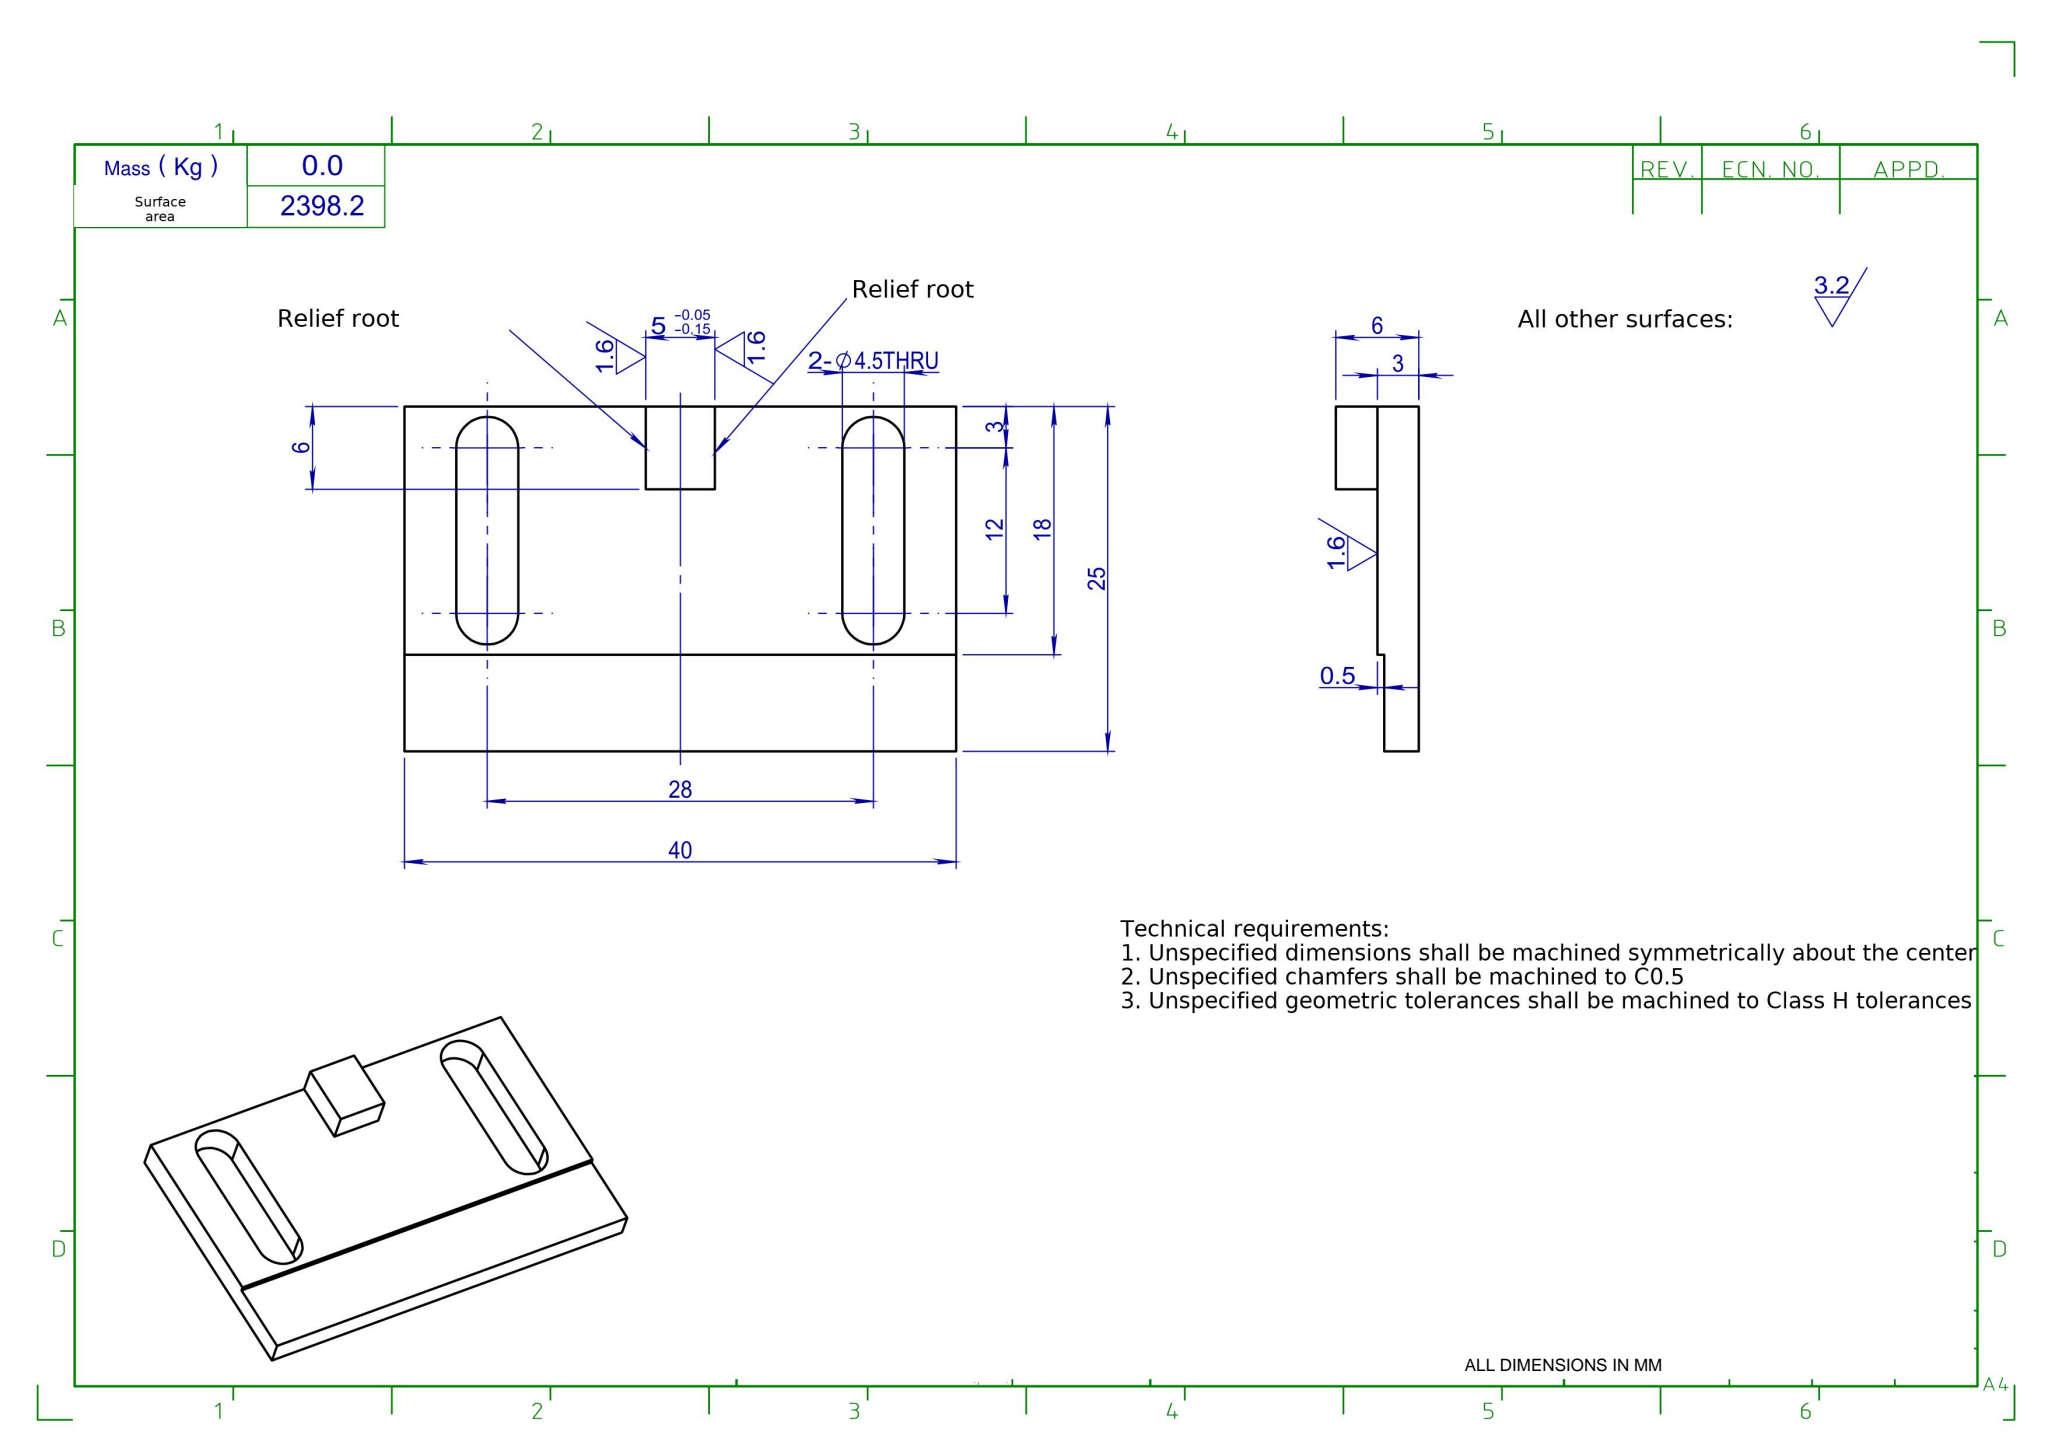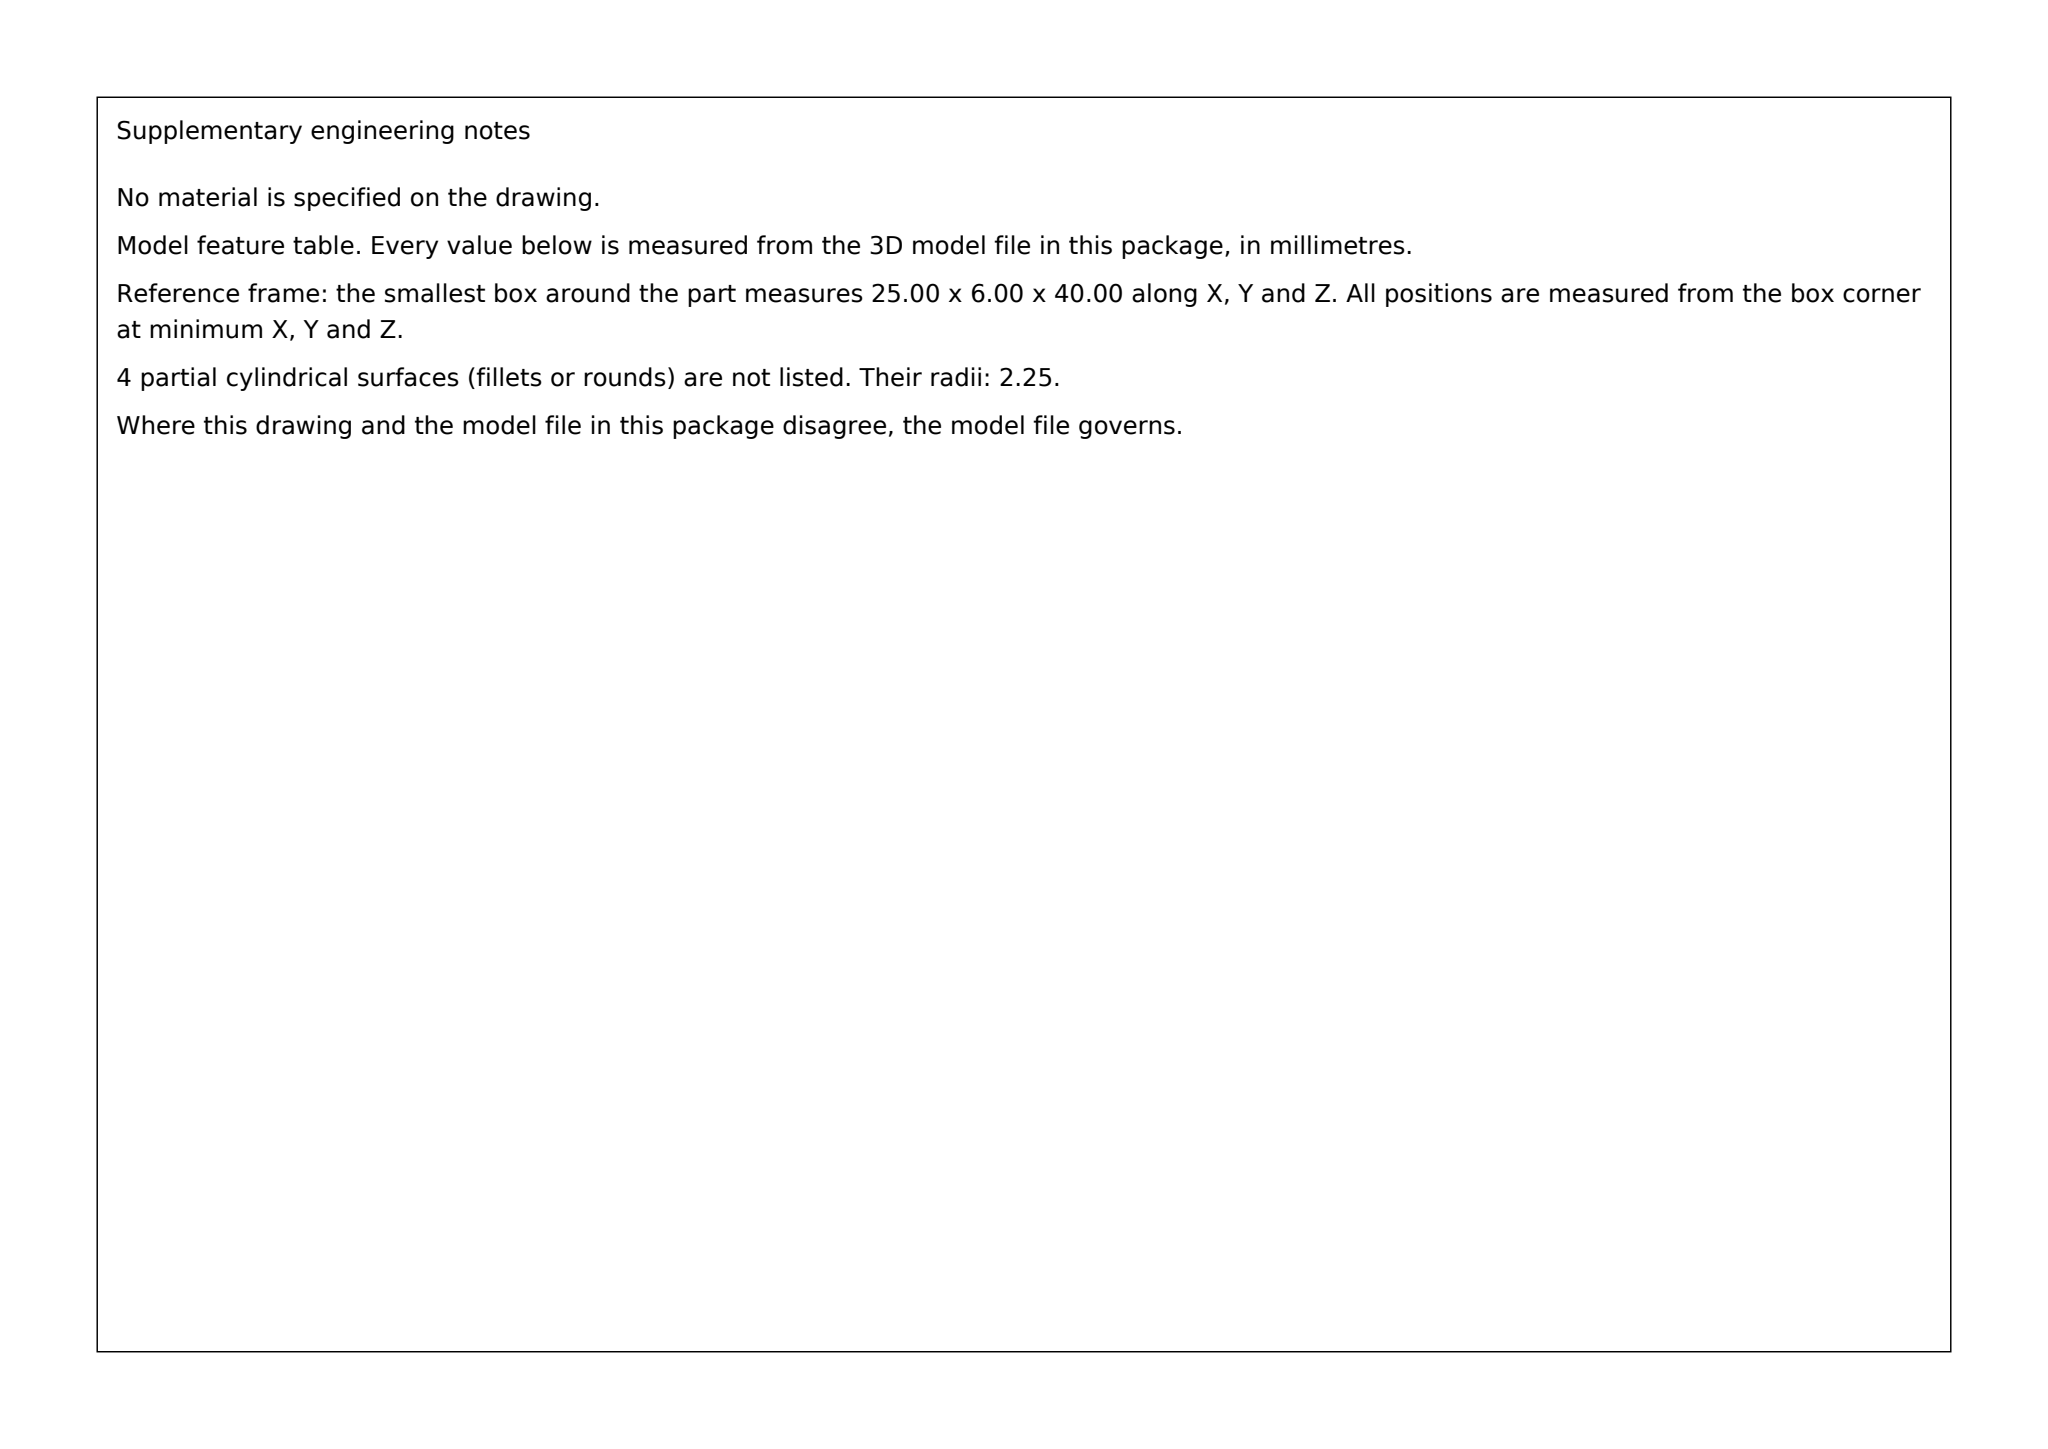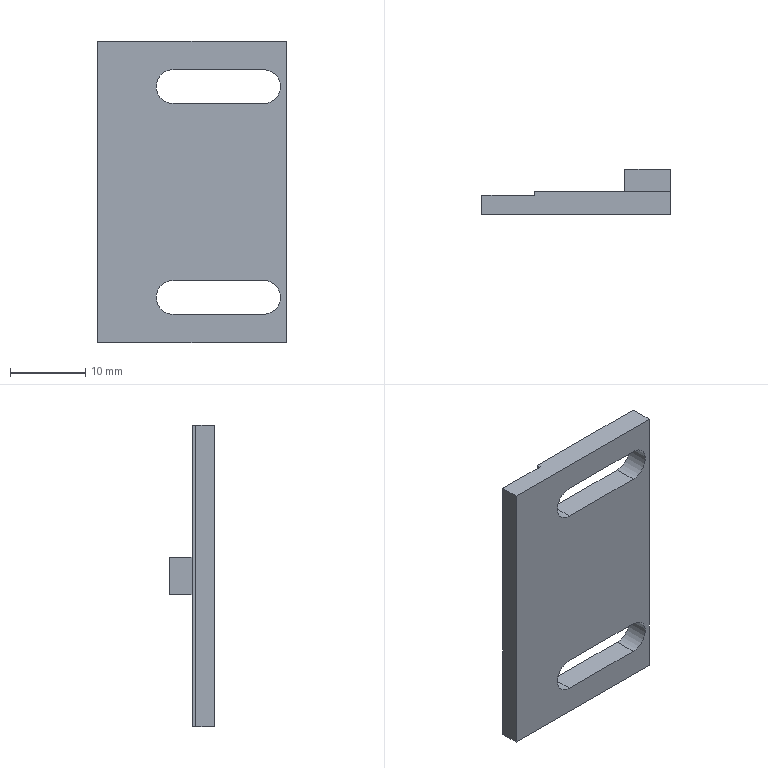Part | SolidWorks | mm | 1 solid | 22 faces | box 25 x 6 x 40 mm | volume 2531 mm3 | plane 16 | cylinder 6 | commonest cylinder face diameters 4.5 x6
build123d program:
from build123d import *

# Parameters (mm, degrees)
SKETCH1_W           = 25
SKETCH1_H           = 3
BOSS_EXTRUDE1_DEPTH = 40
SKETCH2_W           = 7
SKETCH2_H           = 40
CUT_EXTRUDE1_DEPTH  = 0.5
SKETCH3_W           = 6
SKETCH3_H           = 5
BOSS_EXTRUDE2_DEPTH = 3
CUT_EXTRUDE2_DEPTH  = 10


with BuildPart() as part:
    # Sketch1 → Boss-Extrude1 (new body)
    with BuildSketch(Plane.XY):
        Rectangle(SKETCH1_W, SKETCH1_H)
    extrude(amount=BOSS_EXTRUDE1_DEPTH)

    # Sketch2 → Cut-Extrude1 (cut)
    with BuildSketch(Plane(origin=(0, 1.5, 0), x_dir=(1, 0, 0), z_dir=(0, 1, 0))):
        with Locations((-9, -20)):
            Rectangle(SKETCH2_W, SKETCH2_H)
    extrude(amount=-CUT_EXTRUDE1_DEPTH, mode=Mode.SUBTRACT)

    # Sketch3 → Boss-Extrude2 (add)
    with BuildSketch(Plane(origin=(0, 1.5, 0), x_dir=(1, 0, 0), z_dir=(0, 1, 0))):
        with Locations((9.5, -20)):
            Rectangle(SKETCH3_W, SKETCH3_H)
    extrude(amount=BOSS_EXTRUDE2_DEPTH)

    # Sketch4 → Cut-Extrude2 (cut)
    with BuildSketch(Plane(origin=(0, 1.5, 0), x_dir=(1, 0, 0), z_dir=(0, 1, 0))):
        with BuildLine():
            Line((-2.5, -3.75), (9.5, -3.75))
            ThreePointArc((9.5, -3.75), (11.75, -6), (9.5, -8.25))
            Line((9.5, -8.25), (-2.5, -8.25))
            ThreePointArc((-2.5, -8.25), (-4.75, -6), (-2.5, -3.75))
        make_face()
        with BuildLine():
            Line((-2.5, -31.75), (9.5, -31.75))
            ThreePointArc((9.5, -31.75), (11.75, -34), (9.5, -36.25))
            Line((9.5, -36.25), (-2.5, -36.25))
            ThreePointArc((-2.5, -36.25), (-4.75, -34), (-2.5, -31.75))
        make_face()
    extrude(amount=-CUT_EXTRUDE2_DEPTH, mode=Mode.SUBTRACT)


solid = part.part
STEP:
#1=CARTESIAN_POINT('',(-4.75,-1.5,34.));
#2=VERTEX_POINT('',#1);
#3=CARTESIAN_POINT('',(-2.5,-1.5,36.25));
#4=VERTEX_POINT('',#3);
#5=CARTESIAN_POINT('',(-2.5,-1.5,34.));
#6=DIRECTION('',(-0.,1.,0.));
#7=DIRECTION('',(-1.,-0.,0.));
#8=AXIS2_PLACEMENT_3D('',#5,#6,#7);
#9=CIRCLE('',#8,2.25);
#10=EDGE_CURVE('',#2,#4,#9,.T.);
#11=ORIENTED_EDGE('',*,*,#10,.F.);
#12=CARTESIAN_POINT('',(-4.75,1.5,34.));
#13=VERTEX_POINT('',#12);
#14=CARTESIAN_POINT('',(-4.75,-8.5,34.));
#15=DIRECTION('',(-0.,1.,0.));
#16=VECTOR('',#15,1000.);
#17=LINE('',#14,#16);
#18=EDGE_CURVE('',#2,#13,#17,.T.);
#19=ORIENTED_EDGE('',*,*,#18,.T.);
#20=CARTESIAN_POINT('',(-2.5,1.5,36.25));
#21=VERTEX_POINT('',#20);
#22=CARTESIAN_POINT('',(-2.5,1.5,34.));
#23=DIRECTION('',(-0.,1.,0.));
#24=DIRECTION('',(1.,0.,0.));
#25=AXIS2_PLACEMENT_3D('',#22,#23,#24);
#26=CIRCLE('',#25,2.25);
#27=EDGE_CURVE('',#13,#21,#26,.T.);
#28=ORIENTED_EDGE('',*,*,#27,.T.);
#29=CARTESIAN_POINT('',(-2.5,-8.5,36.25));
#30=DIRECTION('',(-0.,1.,0.));
#31=VECTOR('',#30,1000.);
#32=LINE('',#29,#31);
#33=EDGE_CURVE('',#4,#21,#32,.T.);
#34=ORIENTED_EDGE('',*,*,#33,.F.);
#35=EDGE_LOOP('',(#11,#19,#28,#34));
#36=FACE_OUTER_BOUND('',#35,.T.);
#37=CARTESIAN_POINT('',(-2.5,-8.5,34.));
#38=DIRECTION('',(-0.,1.,0.));
#39=DIRECTION('',(-1.,0.,0.));
#40=AXIS2_PLACEMENT_3D('',#37,#38,#39);
#41=CYLINDRICAL_SURFACE('',#40,2.25);
#42=ADVANCED_FACE('',(#36),#41,.F.);
#43=CARTESIAN_POINT('',(-4.75,-1.5,6.));
#44=VERTEX_POINT('',#43);
#45=CARTESIAN_POINT('',(-2.5,-1.5,8.25));
#46=VERTEX_POINT('',#45);
#47=CARTESIAN_POINT('',(-2.5,-1.5,6.));
#48=DIRECTION('',(-0.,1.,0.));
#49=DIRECTION('',(-1.,-0.,0.));
#50=AXIS2_PLACEMENT_3D('',#47,#48,#49);
#51=CIRCLE('',#50,2.25);
#52=EDGE_CURVE('',#44,#46,#51,.T.);
#53=ORIENTED_EDGE('',*,*,#52,.F.);
#54=CARTESIAN_POINT('',(-4.75,1.5,6.));
#55=VERTEX_POINT('',#54);
#56=CARTESIAN_POINT('',(-4.75,-8.5,6.));
#57=DIRECTION('',(-0.,1.,0.));
#58=VECTOR('',#57,1000.);
#59=LINE('',#56,#58);
#60=EDGE_CURVE('',#44,#55,#59,.T.);
#61=ORIENTED_EDGE('',*,*,#60,.T.);
#62=CARTESIAN_POINT('',(-2.5,1.5,8.25));
#63=VERTEX_POINT('',#62);
#64=CARTESIAN_POINT('',(-2.5,1.5,6.));
#65=DIRECTION('',(-0.,1.,0.));
#66=DIRECTION('',(-1.,-0.,0.));
#67=AXIS2_PLACEMENT_3D('',#64,#65,#66);
#68=CIRCLE('',#67,2.25);
#69=EDGE_CURVE('',#55,#63,#68,.T.);
#70=ORIENTED_EDGE('',*,*,#69,.T.);
#71=CARTESIAN_POINT('',(-2.5,-8.5,8.25));
#72=DIRECTION('',(-0.,1.,0.));
#73=VECTOR('',#72,1000.);
#74=LINE('',#71,#73);
#75=EDGE_CURVE('',#46,#63,#74,.T.);
#76=ORIENTED_EDGE('',*,*,#75,.F.);
#77=EDGE_LOOP('',(#53,#61,#70,#76));
#78=FACE_OUTER_BOUND('',#77,.T.);
#79=CARTESIAN_POINT('',(-2.5,-8.5,6.));
#80=DIRECTION('',(-0.,1.,0.));
#81=DIRECTION('',(-1.,0.,0.));
#82=AXIS2_PLACEMENT_3D('',#79,#80,#81);
#83=CYLINDRICAL_SURFACE('',#82,2.25);
#84=ADVANCED_FACE('',(#78),#83,.F.);
#85=CARTESIAN_POINT('',(9.5,1.5,36.25));
#86=VERTEX_POINT('',#85);
#87=CARTESIAN_POINT('',(-2.5,1.5,36.25));
#88=DIRECTION('',(1.,0.,0.));
#89=VECTOR('',#88,1000.);
#90=LINE('',#87,#89);
#91=EDGE_CURVE('',#21,#86,#90,.T.);
#92=ORIENTED_EDGE('',*,*,#91,.F.);
#93=ORIENTED_EDGE('',*,*,#27,.F.);
#94=CARTESIAN_POINT('',(-2.5,1.5,31.75));
#95=VERTEX_POINT('',#94);
#96=CARTESIAN_POINT('',(-2.5,1.5,34.));
#97=DIRECTION('',(-0.,1.,0.));
#98=DIRECTION('',(1.,0.,0.));
#99=AXIS2_PLACEMENT_3D('',#96,#97,#98);
#100=CIRCLE('',#99,2.25);
#101=EDGE_CURVE('',#95,#13,#100,.T.);
#102=ORIENTED_EDGE('',*,*,#101,.F.);
#103=CARTESIAN_POINT('',(9.5,1.5,31.75));
#104=VERTEX_POINT('',#103);
#105=CARTESIAN_POINT('',(-2.5,1.5,31.75));
#106=DIRECTION('',(-1.,-0.,0.));
#107=VECTOR('',#106,1000.);
#108=LINE('',#105,#107);
#109=EDGE_CURVE('',#104,#95,#108,.T.);
#110=ORIENTED_EDGE('',*,*,#109,.F.);
#111=CARTESIAN_POINT('',(9.5,1.5,34.));
#112=DIRECTION('',(-0.,1.,0.));
#113=DIRECTION('',(1.,0.,0.));
#114=AXIS2_PLACEMENT_3D('',#111,#112,#113);
#115=CIRCLE('',#114,2.25);
#116=EDGE_CURVE('',#86,#104,#115,.T.);
#117=ORIENTED_EDGE('',*,*,#116,.F.);
#118=EDGE_LOOP('',(#92,#93,#102,#110,#117));
#119=FACE_BOUND('',#118,.T.);
#120=CARTESIAN_POINT('',(9.5,1.5,8.25));
#121=VERTEX_POINT('',#120);
#122=CARTESIAN_POINT('',(-2.5,1.5,8.25));
#123=DIRECTION('',(1.,0.,0.));
#124=VECTOR('',#123,1000.);
#125=LINE('',#122,#124);
#126=EDGE_CURVE('',#63,#121,#125,.T.);
#127=ORIENTED_EDGE('',*,*,#126,.F.);
#128=ORIENTED_EDGE('',*,*,#69,.F.);
#129=CARTESIAN_POINT('',(-2.5,1.5,3.75));
#130=VERTEX_POINT('',#129);
#131=CARTESIAN_POINT('',(-2.5,1.5,6.));
#132=DIRECTION('',(-0.,1.,0.));
#133=DIRECTION('',(-1.,-0.,0.));
#134=AXIS2_PLACEMENT_3D('',#131,#132,#133);
#135=CIRCLE('',#134,2.25);
#136=EDGE_CURVE('',#130,#55,#135,.T.);
#137=ORIENTED_EDGE('',*,*,#136,.F.);
#138=CARTESIAN_POINT('',(9.5,1.5,3.75));
#139=VERTEX_POINT('',#138);
#140=CARTESIAN_POINT('',(-2.5,1.5,3.75));
#141=DIRECTION('',(-1.,-0.,-0.));
#142=VECTOR('',#141,1000.);
#143=LINE('',#140,#142);
#144=EDGE_CURVE('',#139,#130,#143,.T.);
#145=ORIENTED_EDGE('',*,*,#144,.F.);
#146=CARTESIAN_POINT('',(9.5,1.5,6.));
#147=DIRECTION('',(-0.,1.,0.));
#148=DIRECTION('',(-1.,-0.,0.));
#149=AXIS2_PLACEMENT_3D('',#146,#147,#148);
#150=CIRCLE('',#149,2.25);
#151=EDGE_CURVE('',#121,#139,#150,.T.);
#152=ORIENTED_EDGE('',*,*,#151,.F.);
#153=EDGE_LOOP('',(#127,#128,#137,#145,#152));
#154=FACE_BOUND('',#153,.T.);
#155=CARTESIAN_POINT('',(6.5,1.5,22.5));
#156=VERTEX_POINT('',#155);
#157=CARTESIAN_POINT('',(12.5,1.5,22.5));
#158=VERTEX_POINT('',#157);
#159=CARTESIAN_POINT('',(12.5,1.5,22.5));
#160=DIRECTION('',(1.,0.,-0.));
#161=VECTOR('',#160,1000.);
#162=LINE('',#159,#161);
#163=EDGE_CURVE('',#156,#158,#162,.T.);
#164=ORIENTED_EDGE('',*,*,#163,.F.);
#165=CARTESIAN_POINT('',(6.5,1.5,17.5));
#166=VERTEX_POINT('',#165);
#167=CARTESIAN_POINT('',(6.5,1.5,17.5));
#168=DIRECTION('',(-0.,0.,1.));
#169=VECTOR('',#168,1000.);
#170=LINE('',#167,#169);
#171=EDGE_CURVE('',#166,#156,#170,.T.);
#172=ORIENTED_EDGE('',*,*,#171,.F.);
#173=CARTESIAN_POINT('',(12.5,1.5,17.5));
#174=VERTEX_POINT('',#173);
#175=CARTESIAN_POINT('',(12.5,1.5,17.5));
#176=DIRECTION('',(-1.,-0.,-0.));
#177=VECTOR('',#176,1000.);
#178=LINE('',#175,#177);
#179=EDGE_CURVE('',#174,#166,#178,.T.);
#180=ORIENTED_EDGE('',*,*,#179,.F.);
#181=CARTESIAN_POINT('',(12.5,1.5,0.));
#182=VERTEX_POINT('',#181);
#183=CARTESIAN_POINT('',(12.5,1.5,40.));
#184=DIRECTION('',(0.,0.,-1.));
#185=VECTOR('',#184,1000.);
#186=LINE('',#183,#185);
#187=EDGE_CURVE('',#174,#182,#186,.T.);
#188=ORIENTED_EDGE('',*,*,#187,.T.);
#189=CARTESIAN_POINT('',(-5.5,1.5,0.));
#190=VERTEX_POINT('',#189);
#191=CARTESIAN_POINT('',(12.5,1.5,0.));
#192=DIRECTION('',(-1.,-0.,0.));
#193=VECTOR('',#192,1000.);
#194=LINE('',#191,#193);
#195=EDGE_CURVE('',#182,#190,#194,.T.);
#196=ORIENTED_EDGE('',*,*,#195,.T.);
#197=CARTESIAN_POINT('',(-5.5,1.5,40.));
#198=VERTEX_POINT('',#197);
#199=CARTESIAN_POINT('',(-5.5,1.5,0.));
#200=DIRECTION('',(-0.,0.,-1.));
#201=VECTOR('',#200,1000.);
#202=LINE('',#199,#201);
#203=EDGE_CURVE('',#198,#190,#202,.T.);
#204=ORIENTED_EDGE('',*,*,#203,.F.);
#205=CARTESIAN_POINT('',(12.5,1.5,40.));
#206=VERTEX_POINT('',#205);
#207=CARTESIAN_POINT('',(12.5,1.5,40.));
#208=DIRECTION('',(-1.,-0.,0.));
#209=VECTOR('',#208,1000.);
#210=LINE('',#207,#209);
#211=EDGE_CURVE('',#206,#198,#210,.T.);
#212=ORIENTED_EDGE('',*,*,#211,.F.);
#213=CARTESIAN_POINT('',(12.5,1.5,40.));
#214=DIRECTION('',(0.,0.,-1.));
#215=VECTOR('',#214,1000.);
#216=LINE('',#213,#215);
#217=EDGE_CURVE('',#206,#158,#216,.T.);
#218=ORIENTED_EDGE('',*,*,#217,.T.);
#219=EDGE_LOOP('',(#164,#172,#180,#188,#196,#204,#212,#218));
#220=FACE_OUTER_BOUND('',#219,.T.);
#221=CARTESIAN_POINT('',(12.5,1.5,40.));
#222=DIRECTION('',(0.,-1.,0.));
#223=DIRECTION('',(1.,0.,0.));
#224=AXIS2_PLACEMENT_3D('',#221,#222,#223);
#225=PLANE('',#224);
#226=ADVANCED_FACE('',(#119,#154,#220),#225,.F.);
#227=CARTESIAN_POINT('',(-12.5,1.,0.));
#228=VERTEX_POINT('',#227);
#229=CARTESIAN_POINT('',(-12.5,1.,40.));
#230=VERTEX_POINT('',#229);
#231=CARTESIAN_POINT('',(-12.5,1.,0.));
#232=DIRECTION('',(0.,0.,1.));
#233=VECTOR('',#232,1000.);
#234=LINE('',#231,#233);
#235=EDGE_CURVE('',#228,#230,#234,.T.);
#236=ORIENTED_EDGE('',*,*,#235,.F.);
#237=CARTESIAN_POINT('',(-12.5,-1.5,0.));
#238=VERTEX_POINT('',#237);
#239=CARTESIAN_POINT('',(-12.5,-1.5,0.));
#240=DIRECTION('',(0.,-1.,0.));
#241=VECTOR('',#240,1000.);
#242=LINE('',#239,#241);
#243=EDGE_CURVE('',#228,#238,#242,.T.);
#244=ORIENTED_EDGE('',*,*,#243,.T.);
#245=CARTESIAN_POINT('',(-12.5,-1.5,40.));
#246=VERTEX_POINT('',#245);
#247=CARTESIAN_POINT('',(-12.5,-1.5,40.));
#248=DIRECTION('',(0.,0.,-1.));
#249=VECTOR('',#248,1000.);
#250=LINE('',#247,#249);
#251=EDGE_CURVE('',#246,#238,#250,.T.);
#252=ORIENTED_EDGE('',*,*,#251,.F.);
#253=CARTESIAN_POINT('',(-12.5,-1.5,40.));
#254=DIRECTION('',(0.,-1.,0.));
#255=VECTOR('',#254,1000.);
#256=LINE('',#253,#255);
#257=EDGE_CURVE('',#230,#246,#256,.T.);
#258=ORIENTED_EDGE('',*,*,#257,.F.);
#259=EDGE_LOOP('',(#236,#244,#252,#258));
#260=FACE_OUTER_BOUND('',#259,.T.);
#261=CARTESIAN_POINT('',(-12.5,-1.5,40.));
#262=DIRECTION('',(1.,0.,0.));
#263=DIRECTION('',(0.,0.,-1.));
#264=AXIS2_PLACEMENT_3D('',#261,#262,#263);
#265=PLANE('',#264);
#266=ADVANCED_FACE('',(#260),#265,.F.);
#267=CARTESIAN_POINT('',(9.5,-1.5,31.75));
#268=VERTEX_POINT('',#267);
#269=CARTESIAN_POINT('',(-2.5,-1.5,31.75));
#270=VERTEX_POINT('',#269);
#271=CARTESIAN_POINT('',(12.5,-1.5,31.75));
#272=DIRECTION('',(-1.,-0.,0.));
#273=VECTOR('',#272,1000.);
#274=LINE('',#271,#273);
#275=EDGE_CURVE('',#268,#270,#274,.T.);
#276=ORIENTED_EDGE('',*,*,#275,.T.);
#277=CARTESIAN_POINT('',(-2.5,-1.5,34.));
#278=DIRECTION('',(-0.,1.,0.));
#279=DIRECTION('',(-1.,-0.,0.));
#280=AXIS2_PLACEMENT_3D('',#277,#278,#279);
#281=CIRCLE('',#280,2.25);
#282=EDGE_CURVE('',#270,#2,#281,.T.);
#283=ORIENTED_EDGE('',*,*,#282,.T.);
#284=ORIENTED_EDGE('',*,*,#10,.T.);
#285=CARTESIAN_POINT('',(9.5,-1.5,36.25));
#286=VERTEX_POINT('',#285);
#287=CARTESIAN_POINT('',(12.5,-1.5,36.25));
#288=DIRECTION('',(1.,0.,0.));
#289=VECTOR('',#288,1000.);
#290=LINE('',#287,#289);
#291=EDGE_CURVE('',#4,#286,#290,.T.);
#292=ORIENTED_EDGE('',*,*,#291,.T.);
#293=CARTESIAN_POINT('',(9.5,-1.5,34.));
#294=DIRECTION('',(-0.,1.,0.));
#295=DIRECTION('',(-1.,-0.,0.));
#296=AXIS2_PLACEMENT_3D('',#293,#294,#295);
#297=CIRCLE('',#296,2.25);
#298=EDGE_CURVE('',#286,#268,#297,.T.);
#299=ORIENTED_EDGE('',*,*,#298,.T.);
#300=EDGE_LOOP('',(#276,#283,#284,#292,#299));
#301=FACE_BOUND('',#300,.T.);
#302=CARTESIAN_POINT('',(9.5,-1.5,3.75));
#303=VERTEX_POINT('',#302);
#304=CARTESIAN_POINT('',(-2.5,-1.5,3.75));
#305=VERTEX_POINT('',#304);
#306=CARTESIAN_POINT('',(12.5,-1.5,3.75));
#307=DIRECTION('',(-1.,-0.,-0.));
#308=VECTOR('',#307,1000.);
#309=LINE('',#306,#308);
#310=EDGE_CURVE('',#303,#305,#309,.T.);
#311=ORIENTED_EDGE('',*,*,#310,.T.);
#312=CARTESIAN_POINT('',(-2.5,-1.5,6.));
#313=DIRECTION('',(-0.,1.,0.));
#314=DIRECTION('',(-1.,-0.,0.));
#315=AXIS2_PLACEMENT_3D('',#312,#313,#314);
#316=CIRCLE('',#315,2.25);
#317=EDGE_CURVE('',#305,#44,#316,.T.);
#318=ORIENTED_EDGE('',*,*,#317,.T.);
#319=ORIENTED_EDGE('',*,*,#52,.T.);
#320=CARTESIAN_POINT('',(9.5,-1.5,8.25));
#321=VERTEX_POINT('',#320);
#322=CARTESIAN_POINT('',(12.5,-1.5,8.25));
#323=DIRECTION('',(1.,0.,0.));
#324=VECTOR('',#323,1000.);
#325=LINE('',#322,#324);
#326=EDGE_CURVE('',#46,#321,#325,.T.);
#327=ORIENTED_EDGE('',*,*,#326,.T.);
#328=CARTESIAN_POINT('',(9.5,-1.5,6.));
#329=DIRECTION('',(-0.,1.,0.));
#330=DIRECTION('',(-1.,-0.,0.));
#331=AXIS2_PLACEMENT_3D('',#328,#329,#330);
#332=CIRCLE('',#331,2.25);
#333=EDGE_CURVE('',#321,#303,#332,.T.);
#334=ORIENTED_EDGE('',*,*,#333,.T.);
#335=EDGE_LOOP('',(#311,#318,#319,#327,#334));
#336=FACE_BOUND('',#335,.T.);
#337=CARTESIAN_POINT('',(12.5,-1.5,0.));
#338=VERTEX_POINT('',#337);
#339=CARTESIAN_POINT('',(12.5,-1.5,0.));
#340=DIRECTION('',(1.,0.,0.));
#341=VECTOR('',#340,1000.);
#342=LINE('',#339,#341);
#343=EDGE_CURVE('',#238,#338,#342,.T.);
#344=ORIENTED_EDGE('',*,*,#343,.T.);
#345=CARTESIAN_POINT('',(12.5,-1.5,40.));
#346=VERTEX_POINT('',#345);
#347=CARTESIAN_POINT('',(12.5,-1.5,40.));
#348=DIRECTION('',(0.,0.,-1.));
#349=VECTOR('',#348,1000.);
#350=LINE('',#347,#349);
#351=EDGE_CURVE('',#346,#338,#350,.T.);
#352=ORIENTED_EDGE('',*,*,#351,.F.);
#353=CARTESIAN_POINT('',(12.5,-1.5,40.));
#354=DIRECTION('',(1.,0.,0.));
#355=VECTOR('',#354,1000.);
#356=LINE('',#353,#355);
#357=EDGE_CURVE('',#246,#346,#356,.T.);
#358=ORIENTED_EDGE('',*,*,#357,.F.);
#359=ORIENTED_EDGE('',*,*,#251,.T.);
#360=EDGE_LOOP('',(#344,#352,#358,#359));
#361=FACE_OUTER_BOUND('',#360,.T.);
#362=CARTESIAN_POINT('',(12.5,-1.5,40.));
#363=DIRECTION('',(-0.,1.,0.));
#364=DIRECTION('',(-1.,-0.,0.));
#365=AXIS2_PLACEMENT_3D('',#362,#363,#364);
#366=PLANE('',#365);
#367=ADVANCED_FACE('',(#301,#336,#361),#366,.F.);
#368=CARTESIAN_POINT('',(12.5,-1.5,0.));
#369=DIRECTION('',(0.,1.,0.));
#370=VECTOR('',#369,1000.);
#371=LINE('',#368,#370);
#372=EDGE_CURVE('',#338,#182,#371,.T.);
#373=ORIENTED_EDGE('',*,*,#372,.T.);
#374=ORIENTED_EDGE('',*,*,#187,.F.);
#375=CARTESIAN_POINT('',(12.5,4.5,17.5));
#376=VERTEX_POINT('',#375);
#377=CARTESIAN_POINT('',(12.5,4.5,17.5));
#378=DIRECTION('',(0.,-1.,0.));
#379=VECTOR('',#378,1000.);
#380=LINE('',#377,#379);
#381=EDGE_CURVE('',#376,#174,#380,.T.);
#382=ORIENTED_EDGE('',*,*,#381,.F.);
#383=CARTESIAN_POINT('',(12.5,4.5,22.5));
#384=VERTEX_POINT('',#383);
#385=CARTESIAN_POINT('',(12.5,4.5,17.5));
#386=DIRECTION('',(0.,0.,-1.));
#387=VECTOR('',#386,1000.);
#388=LINE('',#385,#387);
#389=EDGE_CURVE('',#384,#376,#388,.T.);
#390=ORIENTED_EDGE('',*,*,#389,.F.);
#391=CARTESIAN_POINT('',(12.5,4.5,22.5));
#392=DIRECTION('',(0.,-1.,0.));
#393=VECTOR('',#392,1000.);
#394=LINE('',#391,#393);
#395=EDGE_CURVE('',#384,#158,#394,.T.);
#396=ORIENTED_EDGE('',*,*,#395,.T.);
#397=ORIENTED_EDGE('',*,*,#217,.F.);
#398=CARTESIAN_POINT('',(12.5,-1.5,40.));
#399=DIRECTION('',(0.,1.,0.));
#400=VECTOR('',#399,1000.);
#401=LINE('',#398,#400);
#402=EDGE_CURVE('',#346,#206,#401,.T.);
#403=ORIENTED_EDGE('',*,*,#402,.F.);
#404=ORIENTED_EDGE('',*,*,#351,.T.);
#405=EDGE_LOOP('',(#373,#374,#382,#390,#396,#397,#403,#404));
#406=FACE_OUTER_BOUND('',#405,.T.);
#407=CARTESIAN_POINT('',(12.5,-1.5,40.));
#408=DIRECTION('',(-1.,0.,0.));
#409=DIRECTION('',(0.,0.,1.));
#410=AXIS2_PLACEMENT_3D('',#407,#408,#409);
#411=PLANE('',#410);
#412=ADVANCED_FACE('',(#406),#411,.F.);
#413=CARTESIAN_POINT('',(-5.5,1.,40.));
#414=VERTEX_POINT('',#413);
#415=CARTESIAN_POINT('',(-5.5,1.,40.));
#416=DIRECTION('',(-0.,1.,0.));
#417=VECTOR('',#416,1000.);
#418=LINE('',#415,#417);
#419=EDGE_CURVE('',#414,#198,#418,.T.);
#420=ORIENTED_EDGE('',*,*,#419,.F.);
#421=CARTESIAN_POINT('',(-12.5,1.,40.));
#422=DIRECTION('',(1.,0.,0.));
#423=VECTOR('',#422,1000.);
#424=LINE('',#421,#423);
#425=EDGE_CURVE('',#230,#414,#424,.T.);
#426=ORIENTED_EDGE('',*,*,#425,.F.);
#427=ORIENTED_EDGE('',*,*,#257,.T.);
#428=ORIENTED_EDGE('',*,*,#357,.T.);
#429=ORIENTED_EDGE('',*,*,#402,.T.);
#430=ORIENTED_EDGE('',*,*,#211,.T.);
#431=EDGE_LOOP('',(#420,#426,#427,#428,#429,#430));
#432=FACE_OUTER_BOUND('',#431,.T.);
#433=CARTESIAN_POINT('',(0.,0.,40.));
#434=DIRECTION('',(0.,0.,1.));
#435=DIRECTION('',(1.,0.,0.));
#436=AXIS2_PLACEMENT_3D('',#433,#434,#435);
#437=PLANE('',#436);
#438=ADVANCED_FACE('',(#432),#437,.T.);
#439=CARTESIAN_POINT('',(-5.5,1.,0.));
#440=VERTEX_POINT('',#439);
#441=CARTESIAN_POINT('',(-12.5,1.,0.));
#442=DIRECTION('',(-1.,-0.,0.));
#443=VECTOR('',#442,1000.);
#444=LINE('',#441,#443);
#445=EDGE_CURVE('',#440,#228,#444,.T.);
#446=ORIENTED_EDGE('',*,*,#445,.F.);
#447=CARTESIAN_POINT('',(-5.5,1.,0.));
#448=DIRECTION('',(-0.,1.,0.));
#449=VECTOR('',#448,1000.);
#450=LINE('',#447,#449);
#451=EDGE_CURVE('',#440,#190,#450,.T.);
#452=ORIENTED_EDGE('',*,*,#451,.T.);
#453=ORIENTED_EDGE('',*,*,#195,.F.);
#454=ORIENTED_EDGE('',*,*,#372,.F.);
#455=ORIENTED_EDGE('',*,*,#343,.F.);
#456=ORIENTED_EDGE('',*,*,#243,.F.);
#457=EDGE_LOOP('',(#446,#452,#453,#454,#455,#456));
#458=FACE_OUTER_BOUND('',#457,.T.);
#459=CARTESIAN_POINT('',(0.,0.,0.));
#460=DIRECTION('',(0.,0.,1.));
#461=DIRECTION('',(1.,0.,0.));
#462=AXIS2_PLACEMENT_3D('',#459,#460,#461);
#463=PLANE('',#462);
#464=ADVANCED_FACE('',(#458),#463,.F.);
#465=ORIENTED_EDGE('',*,*,#203,.T.);
#466=ORIENTED_EDGE('',*,*,#451,.F.);
#467=CARTESIAN_POINT('',(-5.5,1.,0.));
#468=DIRECTION('',(-0.,0.,-1.));
#469=VECTOR('',#468,1000.);
#470=LINE('',#467,#469);
#471=EDGE_CURVE('',#414,#440,#470,.T.);
#472=ORIENTED_EDGE('',*,*,#471,.F.);
#473=ORIENTED_EDGE('',*,*,#419,.T.);
#474=EDGE_LOOP('',(#465,#466,#472,#473));
#475=FACE_OUTER_BOUND('',#474,.T.);
#476=CARTESIAN_POINT('',(-5.5,1.,0.));
#477=DIRECTION('',(1.,0.,-0.));
#478=DIRECTION('',(-0.,0.,-1.));
#479=AXIS2_PLACEMENT_3D('',#476,#477,#478);
#480=PLANE('',#479);
#481=ADVANCED_FACE('',(#475),#480,.F.);
#482=ORIENTED_EDGE('',*,*,#235,.T.);
#483=ORIENTED_EDGE('',*,*,#425,.T.);
#484=ORIENTED_EDGE('',*,*,#471,.T.);
#485=ORIENTED_EDGE('',*,*,#445,.T.);
#486=EDGE_LOOP('',(#482,#483,#484,#485));
#487=FACE_OUTER_BOUND('',#486,.T.);
#488=CARTESIAN_POINT('',(-0.,1.,0.));
#489=DIRECTION('',(-0.,1.,0.));
#490=DIRECTION('',(-1.,-0.,0.));
#491=AXIS2_PLACEMENT_3D('',#488,#489,#490);
#492=PLANE('',#491);
#493=ADVANCED_FACE('',(#487),#492,.T.);
#494=ORIENTED_EDGE('',*,*,#179,.T.);
#495=CARTESIAN_POINT('',(6.5,4.5,17.5));
#496=VERTEX_POINT('',#495);
#497=CARTESIAN_POINT('',(6.5,4.5,17.5));
#498=DIRECTION('',(0.,-1.,0.));
#499=VECTOR('',#498,1000.);
#500=LINE('',#497,#499);
#501=EDGE_CURVE('',#496,#166,#500,.T.);
#502=ORIENTED_EDGE('',*,*,#501,.F.);
#503=CARTESIAN_POINT('',(12.5,4.5,17.5));
#504=DIRECTION('',(-1.,-0.,-0.));
#505=VECTOR('',#504,1000.);
#506=LINE('',#503,#505);
#507=EDGE_CURVE('',#376,#496,#506,.T.);
#508=ORIENTED_EDGE('',*,*,#507,.F.);
#509=ORIENTED_EDGE('',*,*,#381,.T.);
#510=EDGE_LOOP('',(#494,#502,#508,#509));
#511=FACE_OUTER_BOUND('',#510,.T.);
#512=CARTESIAN_POINT('',(12.5,4.5,17.5));
#513=DIRECTION('',(-0.,-0.,1.));
#514=DIRECTION('',(1.,0.,0.));
#515=AXIS2_PLACEMENT_3D('',#512,#513,#514);
#516=PLANE('',#515);
#517=ADVANCED_FACE('',(#511),#516,.F.);
#518=ORIENTED_EDGE('',*,*,#171,.T.);
#519=CARTESIAN_POINT('',(6.5,4.5,22.5));
#520=VERTEX_POINT('',#519);
#521=CARTESIAN_POINT('',(6.5,4.5,22.5));
#522=DIRECTION('',(0.,-1.,0.));
#523=VECTOR('',#522,1000.);
#524=LINE('',#521,#523);
#525=EDGE_CURVE('',#520,#156,#524,.T.);
#526=ORIENTED_EDGE('',*,*,#525,.F.);
#527=CARTESIAN_POINT('',(6.5,4.5,17.5));
#528=DIRECTION('',(-0.,0.,1.));
#529=VECTOR('',#528,1000.);
#530=LINE('',#527,#529);
#531=EDGE_CURVE('',#496,#520,#530,.T.);
#532=ORIENTED_EDGE('',*,*,#531,.F.);
#533=ORIENTED_EDGE('',*,*,#501,.T.);
#534=EDGE_LOOP('',(#518,#526,#532,#533));
#535=FACE_OUTER_BOUND('',#534,.T.);
#536=CARTESIAN_POINT('',(6.5,4.5,17.5));
#537=DIRECTION('',(1.,0.,0.));
#538=DIRECTION('',(0.,0.,-1.));
#539=AXIS2_PLACEMENT_3D('',#536,#537,#538);
#540=PLANE('',#539);
#541=ADVANCED_FACE('',(#535),#540,.F.);
#542=ORIENTED_EDGE('',*,*,#163,.T.);
#543=ORIENTED_EDGE('',*,*,#395,.F.);
#544=CARTESIAN_POINT('',(12.5,4.5,22.5));
#545=DIRECTION('',(1.,0.,-0.));
#546=VECTOR('',#545,1000.);
#547=LINE('',#544,#546);
#548=EDGE_CURVE('',#520,#384,#547,.T.);
#549=ORIENTED_EDGE('',*,*,#548,.F.);
#550=ORIENTED_EDGE('',*,*,#525,.T.);
#551=EDGE_LOOP('',(#542,#543,#549,#550));
#552=FACE_OUTER_BOUND('',#551,.T.);
#553=CARTESIAN_POINT('',(12.5,4.5,22.5));
#554=DIRECTION('',(-0.,-0.,-1.));
#555=DIRECTION('',(-1.,0.,0.));
#556=AXIS2_PLACEMENT_3D('',#553,#554,#555);
#557=PLANE('',#556);
#558=ADVANCED_FACE('',(#552),#557,.F.);
#559=ORIENTED_EDGE('',*,*,#389,.T.);
#560=ORIENTED_EDGE('',*,*,#507,.T.);
#561=ORIENTED_EDGE('',*,*,#531,.T.);
#562=ORIENTED_EDGE('',*,*,#548,.T.);
#563=EDGE_LOOP('',(#559,#560,#561,#562));
#564=FACE_OUTER_BOUND('',#563,.T.);
#565=CARTESIAN_POINT('',(-0.,4.5,0.));
#566=DIRECTION('',(0.,-1.,0.));
#567=DIRECTION('',(1.,0.,0.));
#568=AXIS2_PLACEMENT_3D('',#565,#566,#567);
#569=PLANE('',#568);
#570=ADVANCED_FACE('',(#564),#569,.F.);
#571=ORIENTED_EDGE('',*,*,#60,.F.);
#572=ORIENTED_EDGE('',*,*,#317,.F.);
#573=CARTESIAN_POINT('',(-2.5,-8.5,3.75));
#574=DIRECTION('',(-0.,1.,0.));
#575=VECTOR('',#574,1000.);
#576=LINE('',#573,#575);
#577=EDGE_CURVE('',#305,#130,#576,.T.);
#578=ORIENTED_EDGE('',*,*,#577,.T.);
#579=ORIENTED_EDGE('',*,*,#136,.T.);
#580=EDGE_LOOP('',(#571,#572,#578,#579));
#581=FACE_OUTER_BOUND('',#580,.T.);
#582=CARTESIAN_POINT('',(-2.5,-8.5,6.));
#583=DIRECTION('',(-0.,1.,0.));
#584=DIRECTION('',(-1.,0.,0.));
#585=AXIS2_PLACEMENT_3D('',#582,#583,#584);
#586=CYLINDRICAL_SURFACE('',#585,2.25);
#587=ADVANCED_FACE('',(#581),#586,.F.);
#588=CARTESIAN_POINT('',(9.5,-8.5,3.75));
#589=DIRECTION('',(-0.,1.,0.));
#590=VECTOR('',#589,1000.);
#591=LINE('',#588,#590);
#592=EDGE_CURVE('',#303,#139,#591,.T.);
#593=ORIENTED_EDGE('',*,*,#592,.T.);
#594=ORIENTED_EDGE('',*,*,#144,.T.);
#595=ORIENTED_EDGE('',*,*,#577,.F.);
#596=ORIENTED_EDGE('',*,*,#310,.F.);
#597=EDGE_LOOP('',(#593,#594,#595,#596));
#598=FACE_OUTER_BOUND('',#597,.T.);
#599=CARTESIAN_POINT('',(-2.5,-8.5,3.75));
#600=DIRECTION('',(0.,0.,-1.));
#601=DIRECTION('',(-1.,0.,-0.));
#602=AXIS2_PLACEMENT_3D('',#599,#600,#601);
#603=PLANE('',#602);
#604=ADVANCED_FACE('',(#598),#603,.F.);
#605=CARTESIAN_POINT('',(9.5,-8.5,8.25));
#606=DIRECTION('',(-0.,1.,0.));
#607=VECTOR('',#606,1000.);
#608=LINE('',#605,#607);
#609=EDGE_CURVE('',#321,#121,#608,.T.);
#610=ORIENTED_EDGE('',*,*,#609,.T.);
#611=ORIENTED_EDGE('',*,*,#151,.T.);
#612=ORIENTED_EDGE('',*,*,#592,.F.);
#613=ORIENTED_EDGE('',*,*,#333,.F.);
#614=EDGE_LOOP('',(#610,#611,#612,#613));
#615=FACE_OUTER_BOUND('',#614,.T.);
#616=CARTESIAN_POINT('',(9.5,-8.5,6.));
#617=DIRECTION('',(-0.,1.,0.));
#618=DIRECTION('',(-1.,0.,0.));
#619=AXIS2_PLACEMENT_3D('',#616,#617,#618);
#620=CYLINDRICAL_SURFACE('',#619,2.25);
#621=ADVANCED_FACE('',(#615),#620,.F.);
#622=ORIENTED_EDGE('',*,*,#75,.T.);
#623=ORIENTED_EDGE('',*,*,#126,.T.);
#624=ORIENTED_EDGE('',*,*,#609,.F.);
#625=ORIENTED_EDGE('',*,*,#326,.F.);
#626=EDGE_LOOP('',(#622,#623,#624,#625));
#627=FACE_OUTER_BOUND('',#626,.T.);
#628=CARTESIAN_POINT('',(-2.5,-8.5,8.25));
#629=DIRECTION('',(0.,0.,1.));
#630=DIRECTION('',(1.,0.,0.));
#631=AXIS2_PLACEMENT_3D('',#628,#629,#630);
#632=PLANE('',#631);
#633=ADVANCED_FACE('',(#627),#632,.F.);
#634=ORIENTED_EDGE('',*,*,#18,.F.);
#635=ORIENTED_EDGE('',*,*,#282,.F.);
#636=CARTESIAN_POINT('',(-2.5,-8.5,31.75));
#637=DIRECTION('',(-0.,1.,0.));
#638=VECTOR('',#637,1000.);
#639=LINE('',#636,#638);
#640=EDGE_CURVE('',#270,#95,#639,.T.);
#641=ORIENTED_EDGE('',*,*,#640,.T.);
#642=ORIENTED_EDGE('',*,*,#101,.T.);
#643=EDGE_LOOP('',(#634,#635,#641,#642));
#644=FACE_OUTER_BOUND('',#643,.T.);
#645=CARTESIAN_POINT('',(-2.5,-8.5,34.));
#646=DIRECTION('',(-0.,1.,0.));
#647=DIRECTION('',(-1.,0.,0.));
#648=AXIS2_PLACEMENT_3D('',#645,#646,#647);
#649=CYLINDRICAL_SURFACE('',#648,2.25);
#650=ADVANCED_FACE('',(#644),#649,.F.);
#651=CARTESIAN_POINT('',(9.5,-8.5,31.75));
#652=DIRECTION('',(-0.,1.,0.));
#653=VECTOR('',#652,1000.);
#654=LINE('',#651,#653);
#655=EDGE_CURVE('',#268,#104,#654,.T.);
#656=ORIENTED_EDGE('',*,*,#655,.T.);
#657=ORIENTED_EDGE('',*,*,#109,.T.);
#658=ORIENTED_EDGE('',*,*,#640,.F.);
#659=ORIENTED_EDGE('',*,*,#275,.F.);
#660=EDGE_LOOP('',(#656,#657,#658,#659));
#661=FACE_OUTER_BOUND('',#660,.T.);
#662=CARTESIAN_POINT('',(-2.5,-8.5,31.75));
#663=DIRECTION('',(-0.,-0.,-1.));
#664=DIRECTION('',(-1.,0.,0.));
#665=AXIS2_PLACEMENT_3D('',#662,#663,#664);
#666=PLANE('',#665);
#667=ADVANCED_FACE('',(#661),#666,.F.);
#668=CARTESIAN_POINT('',(9.5,-8.5,36.25));
#669=DIRECTION('',(-0.,1.,0.));
#670=VECTOR('',#669,1000.);
#671=LINE('',#668,#670);
#672=EDGE_CURVE('',#286,#86,#671,.T.);
#673=ORIENTED_EDGE('',*,*,#672,.T.);
#674=ORIENTED_EDGE('',*,*,#116,.T.);
#675=ORIENTED_EDGE('',*,*,#655,.F.);
#676=ORIENTED_EDGE('',*,*,#298,.F.);
#677=EDGE_LOOP('',(#673,#674,#675,#676));
#678=FACE_OUTER_BOUND('',#677,.T.);
#679=CARTESIAN_POINT('',(9.5,-8.5,34.));
#680=DIRECTION('',(-0.,1.,0.));
#681=DIRECTION('',(-1.,0.,0.));
#682=AXIS2_PLACEMENT_3D('',#679,#680,#681);
#683=CYLINDRICAL_SURFACE('',#682,2.25);
#684=ADVANCED_FACE('',(#678),#683,.F.);
#685=ORIENTED_EDGE('',*,*,#33,.T.);
#686=ORIENTED_EDGE('',*,*,#91,.T.);
#687=ORIENTED_EDGE('',*,*,#672,.F.);
#688=ORIENTED_EDGE('',*,*,#291,.F.);
#689=EDGE_LOOP('',(#685,#686,#687,#688));
#690=FACE_OUTER_BOUND('',#689,.T.);
#691=CARTESIAN_POINT('',(-2.5,-8.5,36.25));
#692=DIRECTION('',(0.,0.,1.));
#693=DIRECTION('',(1.,0.,0.));
#694=AXIS2_PLACEMENT_3D('',#691,#692,#693);
#695=PLANE('',#694);
#696=ADVANCED_FACE('',(#690),#695,.F.);
#697=CLOSED_SHELL('',(#42,#84,#226,#266,#367,#412,#438,#464,#481,#493,#517,#541,#558,#570,#587,#604,#621,#633,#650,#667,#684,#696));
#698=MANIFOLD_SOLID_BREP('',#697);
#699=CARTESIAN_POINT('',(0.,0.,0.));
#700=DIRECTION('',(0.,0.,1.));
#701=DIRECTION('',(1.,0.,0.));
#702=AXIS2_PLACEMENT_3D('',#699,#700,#701);
#703=(LENGTH_UNIT()NAMED_UNIT(*)SI_UNIT(.MILLI.,.METRE.));
#704=UNCERTAINTY_MEASURE_WITH_UNIT(LENGTH_MEASURE(0.00001),#703,'','');
#705=(NAMED_UNIT(*)PLANE_ANGLE_UNIT()SI_UNIT($,.RADIAN.));
#706=(NAMED_UNIT(*)SI_UNIT($,.STERADIAN.)SOLID_ANGLE_UNIT());
#707=(GEOMETRIC_REPRESENTATION_CONTEXT(3)GLOBAL_UNCERTAINTY_ASSIGNED_CONTEXT((#704))GLOBAL_UNIT_ASSIGNED_CONTEXT((#703,#705,#706))REPRESENTATION_CONTEXT('',''));
#708=ADVANCED_BREP_SHAPE_REPRESENTATION('',(#698,#702),#707);